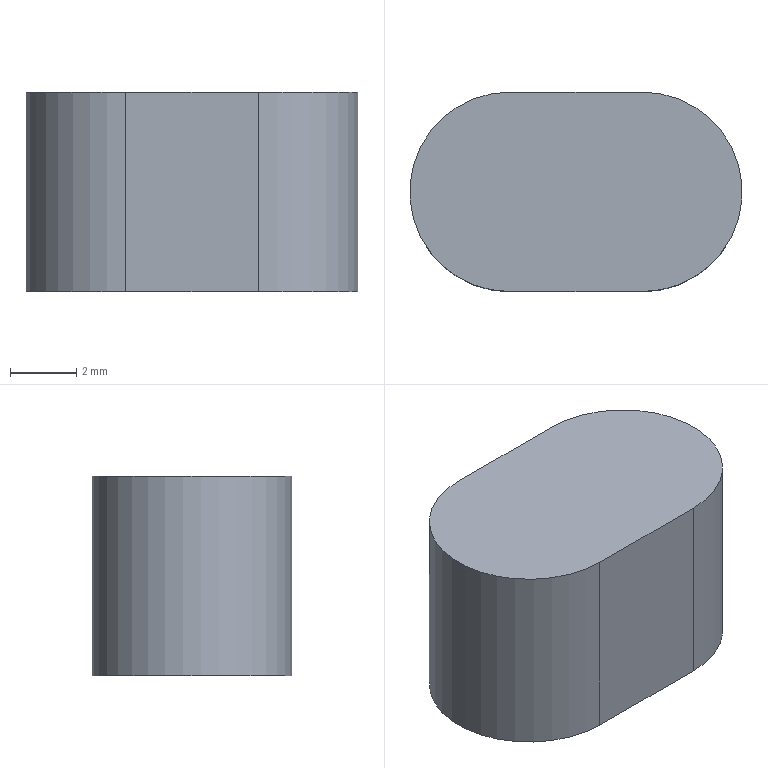Component | NX | KEY_A | 1 solid | 6 faces | box 10 x 6 x 6 mm | volume 314 mm3 | plane 4 | cylinder 2 | commonest cylinder face diameters 6 x2
STEP:
#1=CARTESIAN_POINT('',(0.,0.,0.));
#2=DIRECTION('',(0.,0.,1.));
#3=DIRECTION('',(1.,0.,0.));
#4=AXIS2_PLACEMENT_3D('',#1,#2,#3);
#5=CARTESIAN_POINT('',(95.5,-37.825,69.25));
#6=VERTEX_POINT('',#5);
#7=CARTESIAN_POINT('',(95.5,-43.825,69.25));
#8=VERTEX_POINT('',#7);
#9=CARTESIAN_POINT('',(95.5,-40.825,69.25));
#10=DIRECTION('',(0.,0.,1.));
#11=DIRECTION('',(0.,1.,0.));
#12=AXIS2_PLACEMENT_3D('',#9,#10,#11);
#13=CIRCLE('',#12,3.);
#14=CARTESIAN_POINT('',(97.5,-40.825,69.25));
#15=DIRECTION('',(0.,0.,1.));
#16=DIRECTION('',(0.,1.,0.));
#17=AXIS2_PLACEMENT_3D('',#14,#15,#16);
#18=PLANE('',#17);
#19=CARTESIAN_POINT('',(0.,2.));
#20=DIRECTION('',(1.,0.));
#21=AXIS2_PLACEMENT_2D('',#19,#20);
#22=CIRCLE('',#21,3.);
#23=(GEOMETRIC_REPRESENTATION_CONTEXT(2)PARAMETRIC_REPRESENTATION_CONTEXT()REPRESENTATION_CONTEXT('',''));
#24=DEFINITIONAL_REPRESENTATION('',(#22),#23);
#25=PCURVE('',#18,#24);
#26=CARTESIAN_POINT('',(95.5,-40.825,63.25));
#27=DIRECTION('',(0.,0.,1.));
#28=DIRECTION('',(0.,1.,0.));
#29=AXIS2_PLACEMENT_3D('',#26,#27,#28);
#30=CYLINDRICAL_SURFACE('',#29,3.);
#31=CARTESIAN_POINT('',(0.,6.));
#32=DIRECTION('',(1.,0.));
#33=VECTOR('',#32,1.);
#34=LINE('',#31,#33);
#35=(GEOMETRIC_REPRESENTATION_CONTEXT(2)PARAMETRIC_REPRESENTATION_CONTEXT()REPRESENTATION_CONTEXT('',''));
#36=DEFINITIONAL_REPRESENTATION('',(#34),#35);
#37=PCURVE('',#30,#36);
#38=SURFACE_CURVE('',#13,(#25,#37),.PCURVE_S1.);
#39=EDGE_CURVE('',#6,#8,#38,.T.);
#40=ORIENTED_EDGE('',*,*,#39,.T.);
#41=CARTESIAN_POINT('',(99.5,-43.825,69.25));
#42=VERTEX_POINT('',#41);
#43=CARTESIAN_POINT('',(97.5,-43.825,69.25));
#44=DIRECTION('',(-1.,0.,0.));
#45=VECTOR('',#44,1.);
#46=LINE('',#43,#45);
#47=CARTESIAN_POINT('',(-3.,0.));
#48=DIRECTION('',(0.,1.));
#49=VECTOR('',#48,1.);
#50=LINE('',#47,#49);
#51=(GEOMETRIC_REPRESENTATION_CONTEXT(2)PARAMETRIC_REPRESENTATION_CONTEXT()REPRESENTATION_CONTEXT('',''));
#52=DEFINITIONAL_REPRESENTATION('',(#50),#51);
#53=PCURVE('',#18,#52);
#54=CARTESIAN_POINT('',(97.5,-43.825,63.25));
#55=DIRECTION('',(0.,-1.,0.));
#56=DIRECTION('',(0.,0.,1.));
#57=AXIS2_PLACEMENT_3D('',#54,#55,#56);
#58=PLANE('',#57);
#59=CARTESIAN_POINT('',(6.,0.));
#60=DIRECTION('',(0.,1.));
#61=VECTOR('',#60,1.);
#62=LINE('',#59,#61);
#63=(GEOMETRIC_REPRESENTATION_CONTEXT(2)PARAMETRIC_REPRESENTATION_CONTEXT()REPRESENTATION_CONTEXT('',''));
#64=DEFINITIONAL_REPRESENTATION('',(#62),#63);
#65=PCURVE('',#58,#64);
#66=SURFACE_CURVE('',#46,(#53,#65),.PCURVE_S1.);
#67=EDGE_CURVE('',#42,#8,#66,.T.);
#68=ORIENTED_EDGE('',*,*,#67,.F.);
#69=CARTESIAN_POINT('',(99.5,-37.825,69.25));
#70=VERTEX_POINT('',#69);
#71=CARTESIAN_POINT('',(99.5,-40.825,69.25));
#72=DIRECTION('',(0.,0.,1.));
#73=DIRECTION('',(0.,1.,0.));
#74=AXIS2_PLACEMENT_3D('',#71,#72,#73);
#75=CIRCLE('',#74,3.);
#76=CARTESIAN_POINT('',(0.,-2.));
#77=DIRECTION('',(1.,0.));
#78=AXIS2_PLACEMENT_2D('',#76,#77);
#79=CIRCLE('',#78,3.);
#80=(GEOMETRIC_REPRESENTATION_CONTEXT(2)PARAMETRIC_REPRESENTATION_CONTEXT()REPRESENTATION_CONTEXT('',''));
#81=DEFINITIONAL_REPRESENTATION('',(#79),#80);
#82=PCURVE('',#18,#81);
#83=CARTESIAN_POINT('',(99.5,-40.825,63.25));
#84=DIRECTION('',(0.,0.,1.));
#85=DIRECTION('',(0.,1.,0.));
#86=AXIS2_PLACEMENT_3D('',#83,#84,#85);
#87=CYLINDRICAL_SURFACE('',#86,3.);
#88=CARTESIAN_POINT('',(0.,6.));
#89=DIRECTION('',(1.,0.));
#90=VECTOR('',#89,1.);
#91=LINE('',#88,#90);
#92=(GEOMETRIC_REPRESENTATION_CONTEXT(2)PARAMETRIC_REPRESENTATION_CONTEXT()REPRESENTATION_CONTEXT('',''));
#93=DEFINITIONAL_REPRESENTATION('',(#91),#92);
#94=PCURVE('',#87,#93);
#95=SURFACE_CURVE('',#75,(#82,#94),.PCURVE_S1.);
#96=EDGE_CURVE('',#42,#70,#95,.T.);
#97=ORIENTED_EDGE('',*,*,#96,.T.);
#98=CARTESIAN_POINT('',(97.5,-37.825,69.25));
#99=DIRECTION('',(1.,0.,0.));
#100=VECTOR('',#99,1.);
#101=LINE('',#98,#100);
#102=CARTESIAN_POINT('',(3.,0.));
#103=DIRECTION('',(0.,-1.));
#104=VECTOR('',#103,1.);
#105=LINE('',#102,#104);
#106=(GEOMETRIC_REPRESENTATION_CONTEXT(2)PARAMETRIC_REPRESENTATION_CONTEXT()REPRESENTATION_CONTEXT('',''));
#107=DEFINITIONAL_REPRESENTATION('',(#105),#106);
#108=PCURVE('',#18,#107);
#109=CARTESIAN_POINT('',(97.5,-37.825,63.25));
#110=DIRECTION('',(0.,1.,0.));
#111=DIRECTION('',(0.,0.,-1.));
#112=AXIS2_PLACEMENT_3D('',#109,#110,#111);
#113=PLANE('',#112);
#114=CARTESIAN_POINT('',(-6.,0.));
#115=DIRECTION('',(0.,-1.));
#116=VECTOR('',#115,1.);
#117=LINE('',#114,#116);
#118=(GEOMETRIC_REPRESENTATION_CONTEXT(2)PARAMETRIC_REPRESENTATION_CONTEXT()REPRESENTATION_CONTEXT('',''));
#119=DEFINITIONAL_REPRESENTATION('',(#117),#118);
#120=PCURVE('',#113,#119);
#121=SURFACE_CURVE('',#101,(#108,#120),.PCURVE_S1.);
#122=EDGE_CURVE('',#6,#70,#121,.T.);
#123=ORIENTED_EDGE('',*,*,#122,.F.);
#124=EDGE_LOOP('',(#40,#68,#97,#123));
#125=FACE_BOUND('',#124,.T.);
#126=ADVANCED_FACE('',(#125),#18,.T.);
#127=ORIENTED_EDGE('',*,*,#67,.T.);
#128=CARTESIAN_POINT('',(95.5,-43.825,63.25));
#129=VERTEX_POINT('',#128);
#130=CARTESIAN_POINT('',(95.5,-43.825,63.25));
#131=DIRECTION('',(0.,0.,-1.));
#132=VECTOR('',#131,1.);
#133=LINE('',#130,#132);
#134=CARTESIAN_POINT('',(0.,2.));
#135=DIRECTION('',(-1.,0.));
#136=VECTOR('',#135,1.);
#137=LINE('',#134,#136);
#138=(GEOMETRIC_REPRESENTATION_CONTEXT(2)PARAMETRIC_REPRESENTATION_CONTEXT()REPRESENTATION_CONTEXT('',''));
#139=DEFINITIONAL_REPRESENTATION('',(#137),#138);
#140=PCURVE('',#58,#139);
#141=CARTESIAN_POINT('',(3.142,0.));
#142=DIRECTION('',(0.,-1.));
#143=VECTOR('',#142,1.);
#144=LINE('',#141,#143);
#145=(GEOMETRIC_REPRESENTATION_CONTEXT(2)PARAMETRIC_REPRESENTATION_CONTEXT()REPRESENTATION_CONTEXT('',''));
#146=DEFINITIONAL_REPRESENTATION('',(#144),#145);
#147=PCURVE('',#30,#146);
#148=SURFACE_CURVE('',#133,(#140,#147),.PCURVE_S1.);
#149=EDGE_CURVE('',#8,#129,#148,.T.);
#150=ORIENTED_EDGE('',*,*,#149,.T.);
#151=CARTESIAN_POINT('',(99.5,-43.825,63.25));
#152=VERTEX_POINT('',#151);
#153=CARTESIAN_POINT('',(97.5,-43.825,63.25));
#154=DIRECTION('',(1.,0.,0.));
#155=VECTOR('',#154,1.);
#156=LINE('',#153,#155);
#157=CARTESIAN_POINT('',(0.,0.));
#158=DIRECTION('',(0.,-1.));
#159=VECTOR('',#158,1.);
#160=LINE('',#157,#159);
#161=(GEOMETRIC_REPRESENTATION_CONTEXT(2)PARAMETRIC_REPRESENTATION_CONTEXT()REPRESENTATION_CONTEXT('',''));
#162=DEFINITIONAL_REPRESENTATION('',(#160),#161);
#163=PCURVE('',#58,#162);
#164=CARTESIAN_POINT('',(97.5,-40.825,63.25));
#165=DIRECTION('',(0.,0.,-1.));
#166=DIRECTION('',(0.,-1.,0.));
#167=AXIS2_PLACEMENT_3D('',#164,#165,#166);
#168=PLANE('',#167);
#169=CARTESIAN_POINT('',(3.,0.));
#170=DIRECTION('',(0.,-1.));
#171=VECTOR('',#170,1.);
#172=LINE('',#169,#171);
#173=(GEOMETRIC_REPRESENTATION_CONTEXT(2)PARAMETRIC_REPRESENTATION_CONTEXT()REPRESENTATION_CONTEXT('',''));
#174=DEFINITIONAL_REPRESENTATION('',(#172),#173);
#175=PCURVE('',#168,#174);
#176=SURFACE_CURVE('',#156,(#163,#175),.PCURVE_S1.);
#177=EDGE_CURVE('',#129,#152,#176,.T.);
#178=ORIENTED_EDGE('',*,*,#177,.T.);
#179=CARTESIAN_POINT('',(99.5,-43.825,63.25));
#180=DIRECTION('',(0.,0.,1.));
#181=VECTOR('',#180,1.);
#182=LINE('',#179,#181);
#183=CARTESIAN_POINT('',(0.,-2.));
#184=DIRECTION('',(1.,0.));
#185=VECTOR('',#184,1.);
#186=LINE('',#183,#185);
#187=(GEOMETRIC_REPRESENTATION_CONTEXT(2)PARAMETRIC_REPRESENTATION_CONTEXT()REPRESENTATION_CONTEXT('',''));
#188=DEFINITIONAL_REPRESENTATION('',(#186),#187);
#189=PCURVE('',#58,#188);
#190=CARTESIAN_POINT('',(3.142,0.));
#191=DIRECTION('',(0.,1.));
#192=VECTOR('',#191,1.);
#193=LINE('',#190,#192);
#194=(GEOMETRIC_REPRESENTATION_CONTEXT(2)PARAMETRIC_REPRESENTATION_CONTEXT()REPRESENTATION_CONTEXT('',''));
#195=DEFINITIONAL_REPRESENTATION('',(#193),#194);
#196=PCURVE('',#87,#195);
#197=SURFACE_CURVE('',#182,(#189,#196),.PCURVE_S1.);
#198=EDGE_CURVE('',#152,#42,#197,.T.);
#199=ORIENTED_EDGE('',*,*,#198,.T.);
#200=EDGE_LOOP('',(#127,#150,#178,#199));
#201=FACE_BOUND('',#200,.T.);
#202=ADVANCED_FACE('',(#201),#58,.T.);
#203=ORIENTED_EDGE('',*,*,#177,.F.);
#204=CARTESIAN_POINT('',(95.5,-37.825,63.25));
#205=VERTEX_POINT('',#204);
#206=CARTESIAN_POINT('',(95.5,-40.825,63.25));
#207=DIRECTION('',(0.,0.,-1.));
#208=DIRECTION('',(0.,-1.,0.));
#209=AXIS2_PLACEMENT_3D('',#206,#207,#208);
#210=CIRCLE('',#209,3.);
#211=CARTESIAN_POINT('',(0.,2.));
#212=DIRECTION('',(1.,0.));
#213=AXIS2_PLACEMENT_2D('',#211,#212);
#214=CIRCLE('',#213,3.);
#215=(GEOMETRIC_REPRESENTATION_CONTEXT(2)PARAMETRIC_REPRESENTATION_CONTEXT()REPRESENTATION_CONTEXT('',''));
#216=DEFINITIONAL_REPRESENTATION('',(#214),#215);
#217=PCURVE('',#168,#216);
#218=CARTESIAN_POINT('',(3.142,0.));
#219=DIRECTION('',(-1.,0.));
#220=VECTOR('',#219,1.);
#221=LINE('',#218,#220);
#222=(GEOMETRIC_REPRESENTATION_CONTEXT(2)PARAMETRIC_REPRESENTATION_CONTEXT()REPRESENTATION_CONTEXT('',''));
#223=DEFINITIONAL_REPRESENTATION('',(#221),#222);
#224=PCURVE('',#30,#223);
#225=SURFACE_CURVE('',#210,(#217,#224),.PCURVE_S1.);
#226=EDGE_CURVE('',#129,#205,#225,.T.);
#227=ORIENTED_EDGE('',*,*,#226,.T.);
#228=CARTESIAN_POINT('',(99.5,-37.825,63.25));
#229=VERTEX_POINT('',#228);
#230=CARTESIAN_POINT('',(97.5,-37.825,63.25));
#231=DIRECTION('',(-1.,0.,0.));
#232=VECTOR('',#231,1.);
#233=LINE('',#230,#232);
#234=CARTESIAN_POINT('',(-3.,0.));
#235=DIRECTION('',(0.,1.));
#236=VECTOR('',#235,1.);
#237=LINE('',#234,#236);
#238=(GEOMETRIC_REPRESENTATION_CONTEXT(2)PARAMETRIC_REPRESENTATION_CONTEXT()REPRESENTATION_CONTEXT('',''));
#239=DEFINITIONAL_REPRESENTATION('',(#237),#238);
#240=PCURVE('',#168,#239);
#241=CARTESIAN_POINT('',(0.,0.));
#242=DIRECTION('',(0.,1.));
#243=VECTOR('',#242,1.);
#244=LINE('',#241,#243);
#245=(GEOMETRIC_REPRESENTATION_CONTEXT(2)PARAMETRIC_REPRESENTATION_CONTEXT()REPRESENTATION_CONTEXT('',''));
#246=DEFINITIONAL_REPRESENTATION('',(#244),#245);
#247=PCURVE('',#113,#246);
#248=SURFACE_CURVE('',#233,(#240,#247),.PCURVE_S1.);
#249=EDGE_CURVE('',#229,#205,#248,.T.);
#250=ORIENTED_EDGE('',*,*,#249,.F.);
#251=CARTESIAN_POINT('',(99.5,-40.825,63.25));
#252=DIRECTION('',(0.,0.,-1.));
#253=DIRECTION('',(0.,-1.,0.));
#254=AXIS2_PLACEMENT_3D('',#251,#252,#253);
#255=CIRCLE('',#254,3.);
#256=CARTESIAN_POINT('',(0.,-2.));
#257=DIRECTION('',(1.,0.));
#258=AXIS2_PLACEMENT_2D('',#256,#257);
#259=CIRCLE('',#258,3.);
#260=(GEOMETRIC_REPRESENTATION_CONTEXT(2)PARAMETRIC_REPRESENTATION_CONTEXT()REPRESENTATION_CONTEXT('',''));
#261=DEFINITIONAL_REPRESENTATION('',(#259),#260);
#262=PCURVE('',#168,#261);
#263=CARTESIAN_POINT('',(9.425,0.));
#264=DIRECTION('',(-1.,0.));
#265=VECTOR('',#264,1.);
#266=LINE('',#263,#265);
#267=(GEOMETRIC_REPRESENTATION_CONTEXT(2)PARAMETRIC_REPRESENTATION_CONTEXT()REPRESENTATION_CONTEXT('',''));
#268=DEFINITIONAL_REPRESENTATION('',(#266),#267);
#269=PCURVE('',#87,#268);
#270=SURFACE_CURVE('',#255,(#262,#269),.PCURVE_S1.);
#271=EDGE_CURVE('',#229,#152,#270,.T.);
#272=ORIENTED_EDGE('',*,*,#271,.T.);
#273=EDGE_LOOP('',(#203,#227,#250,#272));
#274=FACE_BOUND('',#273,.T.);
#275=ADVANCED_FACE('',(#274),#168,.T.);
#276=ORIENTED_EDGE('',*,*,#249,.T.);
#277=CARTESIAN_POINT('',(95.5,-37.825,63.25));
#278=DIRECTION('',(0.,0.,1.));
#279=VECTOR('',#278,1.);
#280=LINE('',#277,#279);
#281=CARTESIAN_POINT('',(0.,2.));
#282=DIRECTION('',(-1.,0.));
#283=VECTOR('',#282,1.);
#284=LINE('',#281,#283);
#285=(GEOMETRIC_REPRESENTATION_CONTEXT(2)PARAMETRIC_REPRESENTATION_CONTEXT()REPRESENTATION_CONTEXT('',''));
#286=DEFINITIONAL_REPRESENTATION('',(#284),#285);
#287=PCURVE('',#113,#286);
#288=CARTESIAN_POINT('',(0.,0.));
#289=DIRECTION('',(0.,1.));
#290=VECTOR('',#289,1.);
#291=LINE('',#288,#290);
#292=(GEOMETRIC_REPRESENTATION_CONTEXT(2)PARAMETRIC_REPRESENTATION_CONTEXT()REPRESENTATION_CONTEXT('',''));
#293=DEFINITIONAL_REPRESENTATION('',(#291),#292);
#294=PCURVE('',#30,#293);
#295=SURFACE_CURVE('',#280,(#287,#294),.PCURVE_S1.);
#296=EDGE_CURVE('',#205,#6,#295,.T.);
#297=ORIENTED_EDGE('',*,*,#296,.T.);
#298=ORIENTED_EDGE('',*,*,#122,.T.);
#299=CARTESIAN_POINT('',(99.5,-37.825,63.25));
#300=DIRECTION('',(0.,0.,-1.));
#301=VECTOR('',#300,1.);
#302=LINE('',#299,#301);
#303=CARTESIAN_POINT('',(0.,-2.));
#304=DIRECTION('',(1.,0.));
#305=VECTOR('',#304,1.);
#306=LINE('',#303,#305);
#307=(GEOMETRIC_REPRESENTATION_CONTEXT(2)PARAMETRIC_REPRESENTATION_CONTEXT()REPRESENTATION_CONTEXT('',''));
#308=DEFINITIONAL_REPRESENTATION('',(#306),#307);
#309=PCURVE('',#113,#308);
#310=CARTESIAN_POINT('',(6.283,0.));
#311=DIRECTION('',(0.,-1.));
#312=VECTOR('',#311,1.);
#313=LINE('',#310,#312);
#314=(GEOMETRIC_REPRESENTATION_CONTEXT(2)PARAMETRIC_REPRESENTATION_CONTEXT()REPRESENTATION_CONTEXT('',''));
#315=DEFINITIONAL_REPRESENTATION('',(#313),#314);
#316=PCURVE('',#87,#315);
#317=SURFACE_CURVE('',#302,(#309,#316),.PCURVE_S1.);
#318=EDGE_CURVE('',#70,#229,#317,.T.);
#319=ORIENTED_EDGE('',*,*,#318,.T.);
#320=EDGE_LOOP('',(#276,#297,#298,#319));
#321=FACE_BOUND('',#320,.T.);
#322=ADVANCED_FACE('',(#321),#113,.T.);
#323=ORIENTED_EDGE('',*,*,#296,.F.);
#324=ORIENTED_EDGE('',*,*,#226,.F.);
#325=ORIENTED_EDGE('',*,*,#149,.F.);
#326=ORIENTED_EDGE('',*,*,#39,.F.);
#327=EDGE_LOOP('',(#323,#324,#325,#326));
#328=FACE_BOUND('',#327,.T.);
#329=ADVANCED_FACE('',(#328),#30,.T.);
#330=ORIENTED_EDGE('',*,*,#96,.F.);
#331=ORIENTED_EDGE('',*,*,#198,.F.);
#332=ORIENTED_EDGE('',*,*,#271,.F.);
#333=ORIENTED_EDGE('',*,*,#318,.F.);
#334=EDGE_LOOP('',(#330,#331,#332,#333));
#335=FACE_BOUND('',#334,.T.);
#336=ADVANCED_FACE('',(#335),#87,.T.);
#337=CLOSED_SHELL('',(#126,#202,#275,#322,#329,#336));
#338=MANIFOLD_SOLID_BREP('',#337);
#339=(LENGTH_UNIT()NAMED_UNIT(*)SI_UNIT(.MILLI.,.METRE.));
#340=UNCERTAINTY_MEASURE_WITH_UNIT(LENGTH_MEASURE(0.0000001),#339,'','');
#341=(NAMED_UNIT(*)PLANE_ANGLE_UNIT()SI_UNIT($,.RADIAN.));
#342=(NAMED_UNIT(*)SI_UNIT($,.STERADIAN.)SOLID_ANGLE_UNIT());
#343=(GEOMETRIC_REPRESENTATION_CONTEXT(3)GLOBAL_UNCERTAINTY_ASSIGNED_CONTEXT((#340))GLOBAL_UNIT_ASSIGNED_CONTEXT((#339,#341,#342))REPRESENTATION_CONTEXT('',''));
#344=ADVANCED_BREP_SHAPE_REPRESENTATION('',(#4,#338),#343);